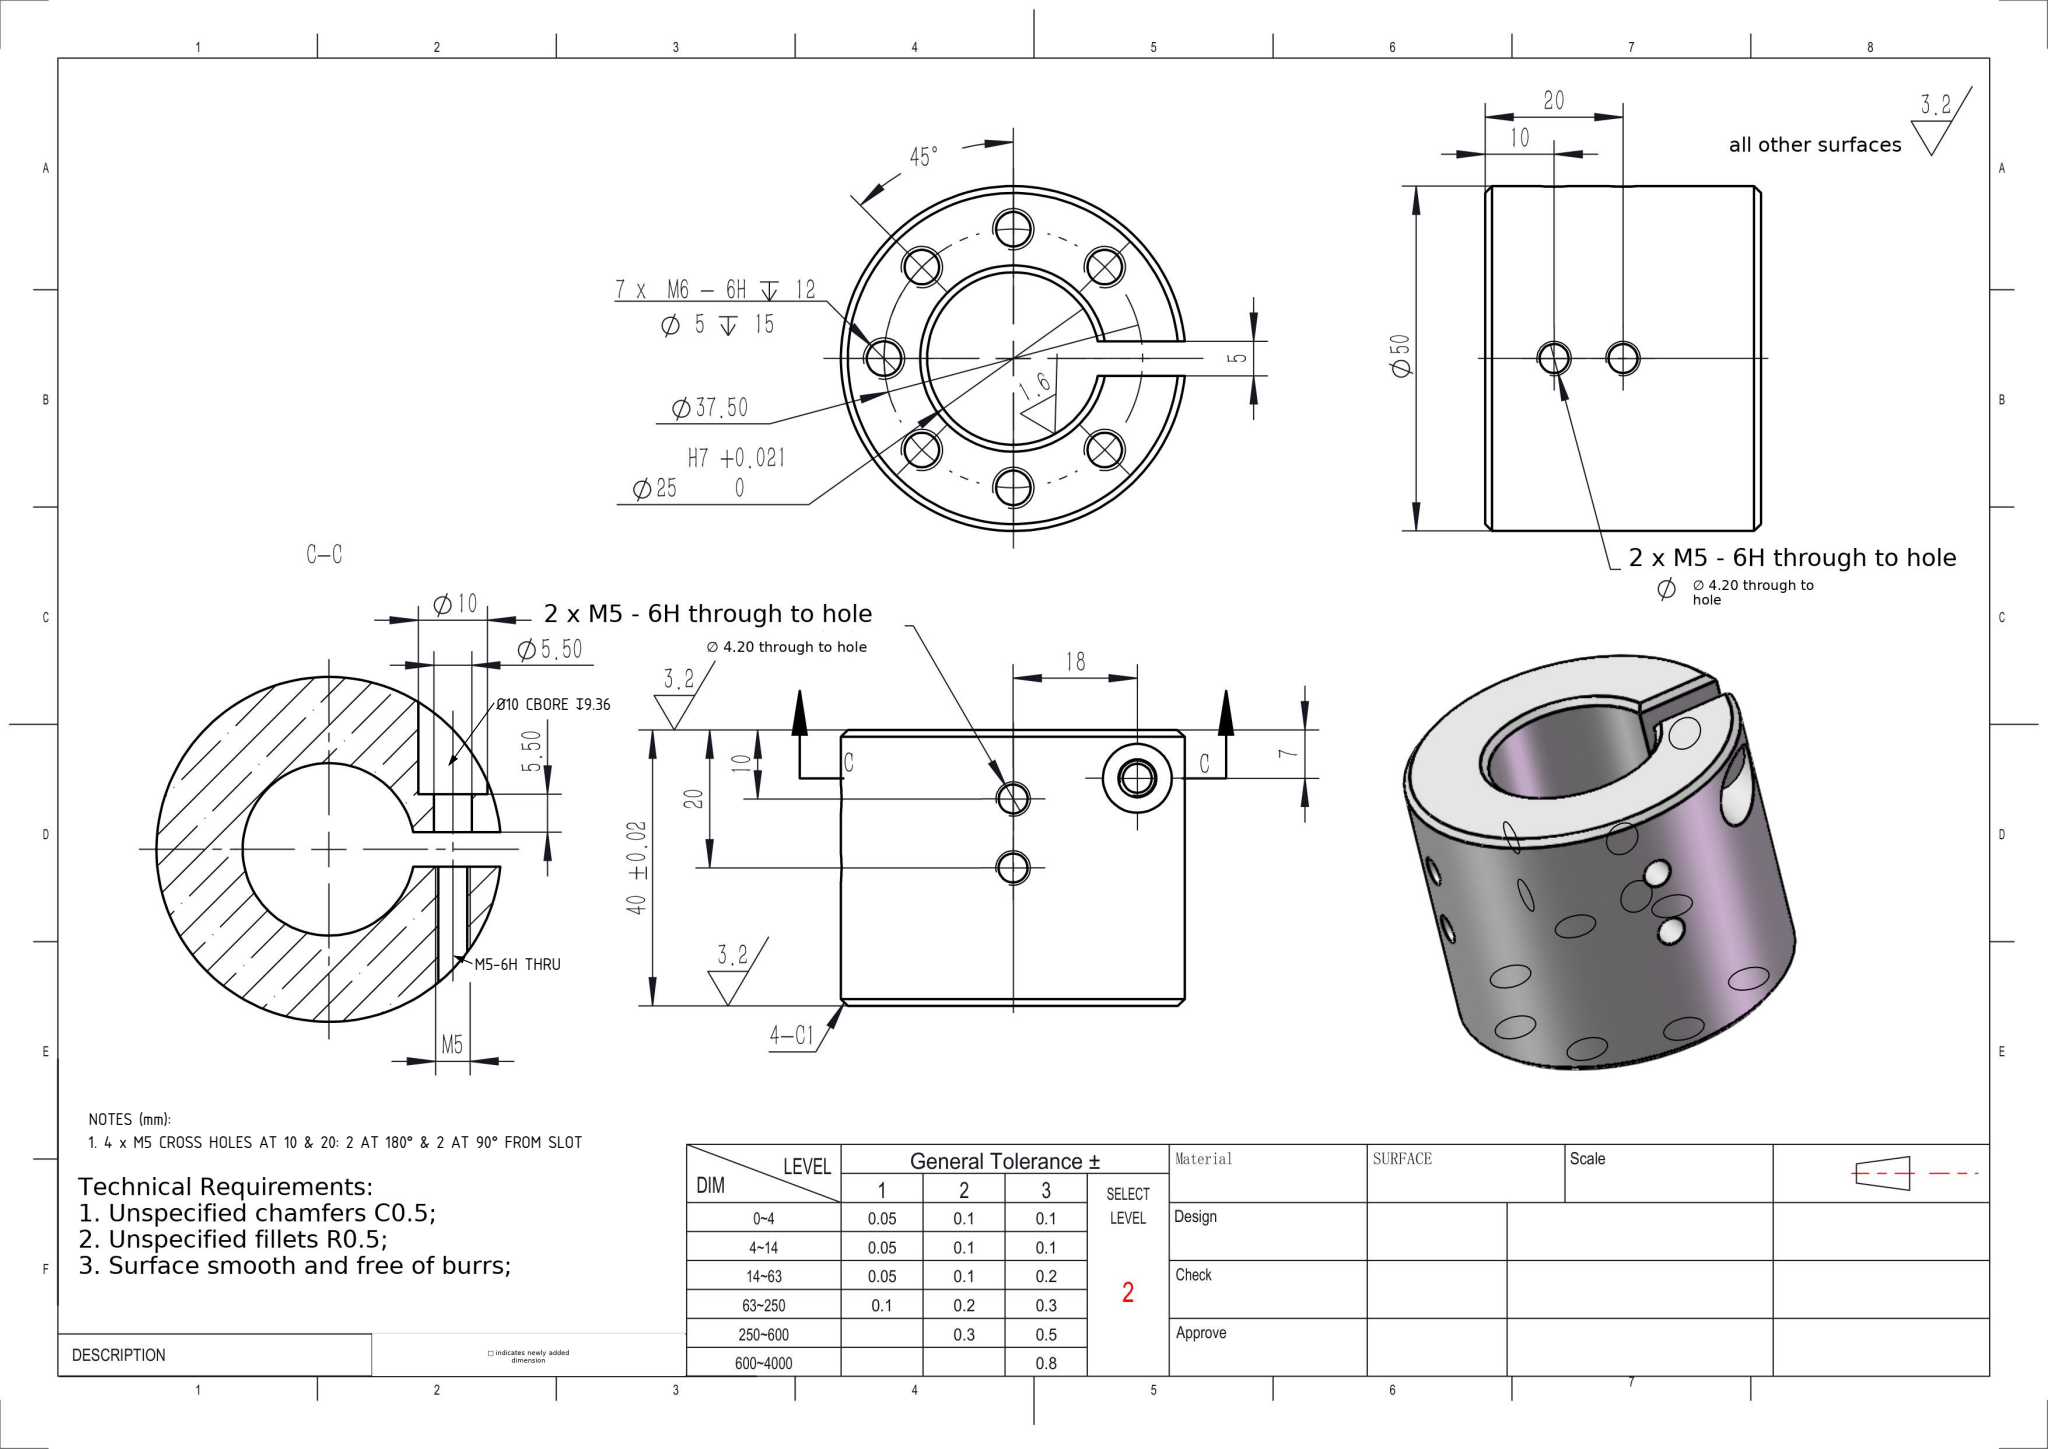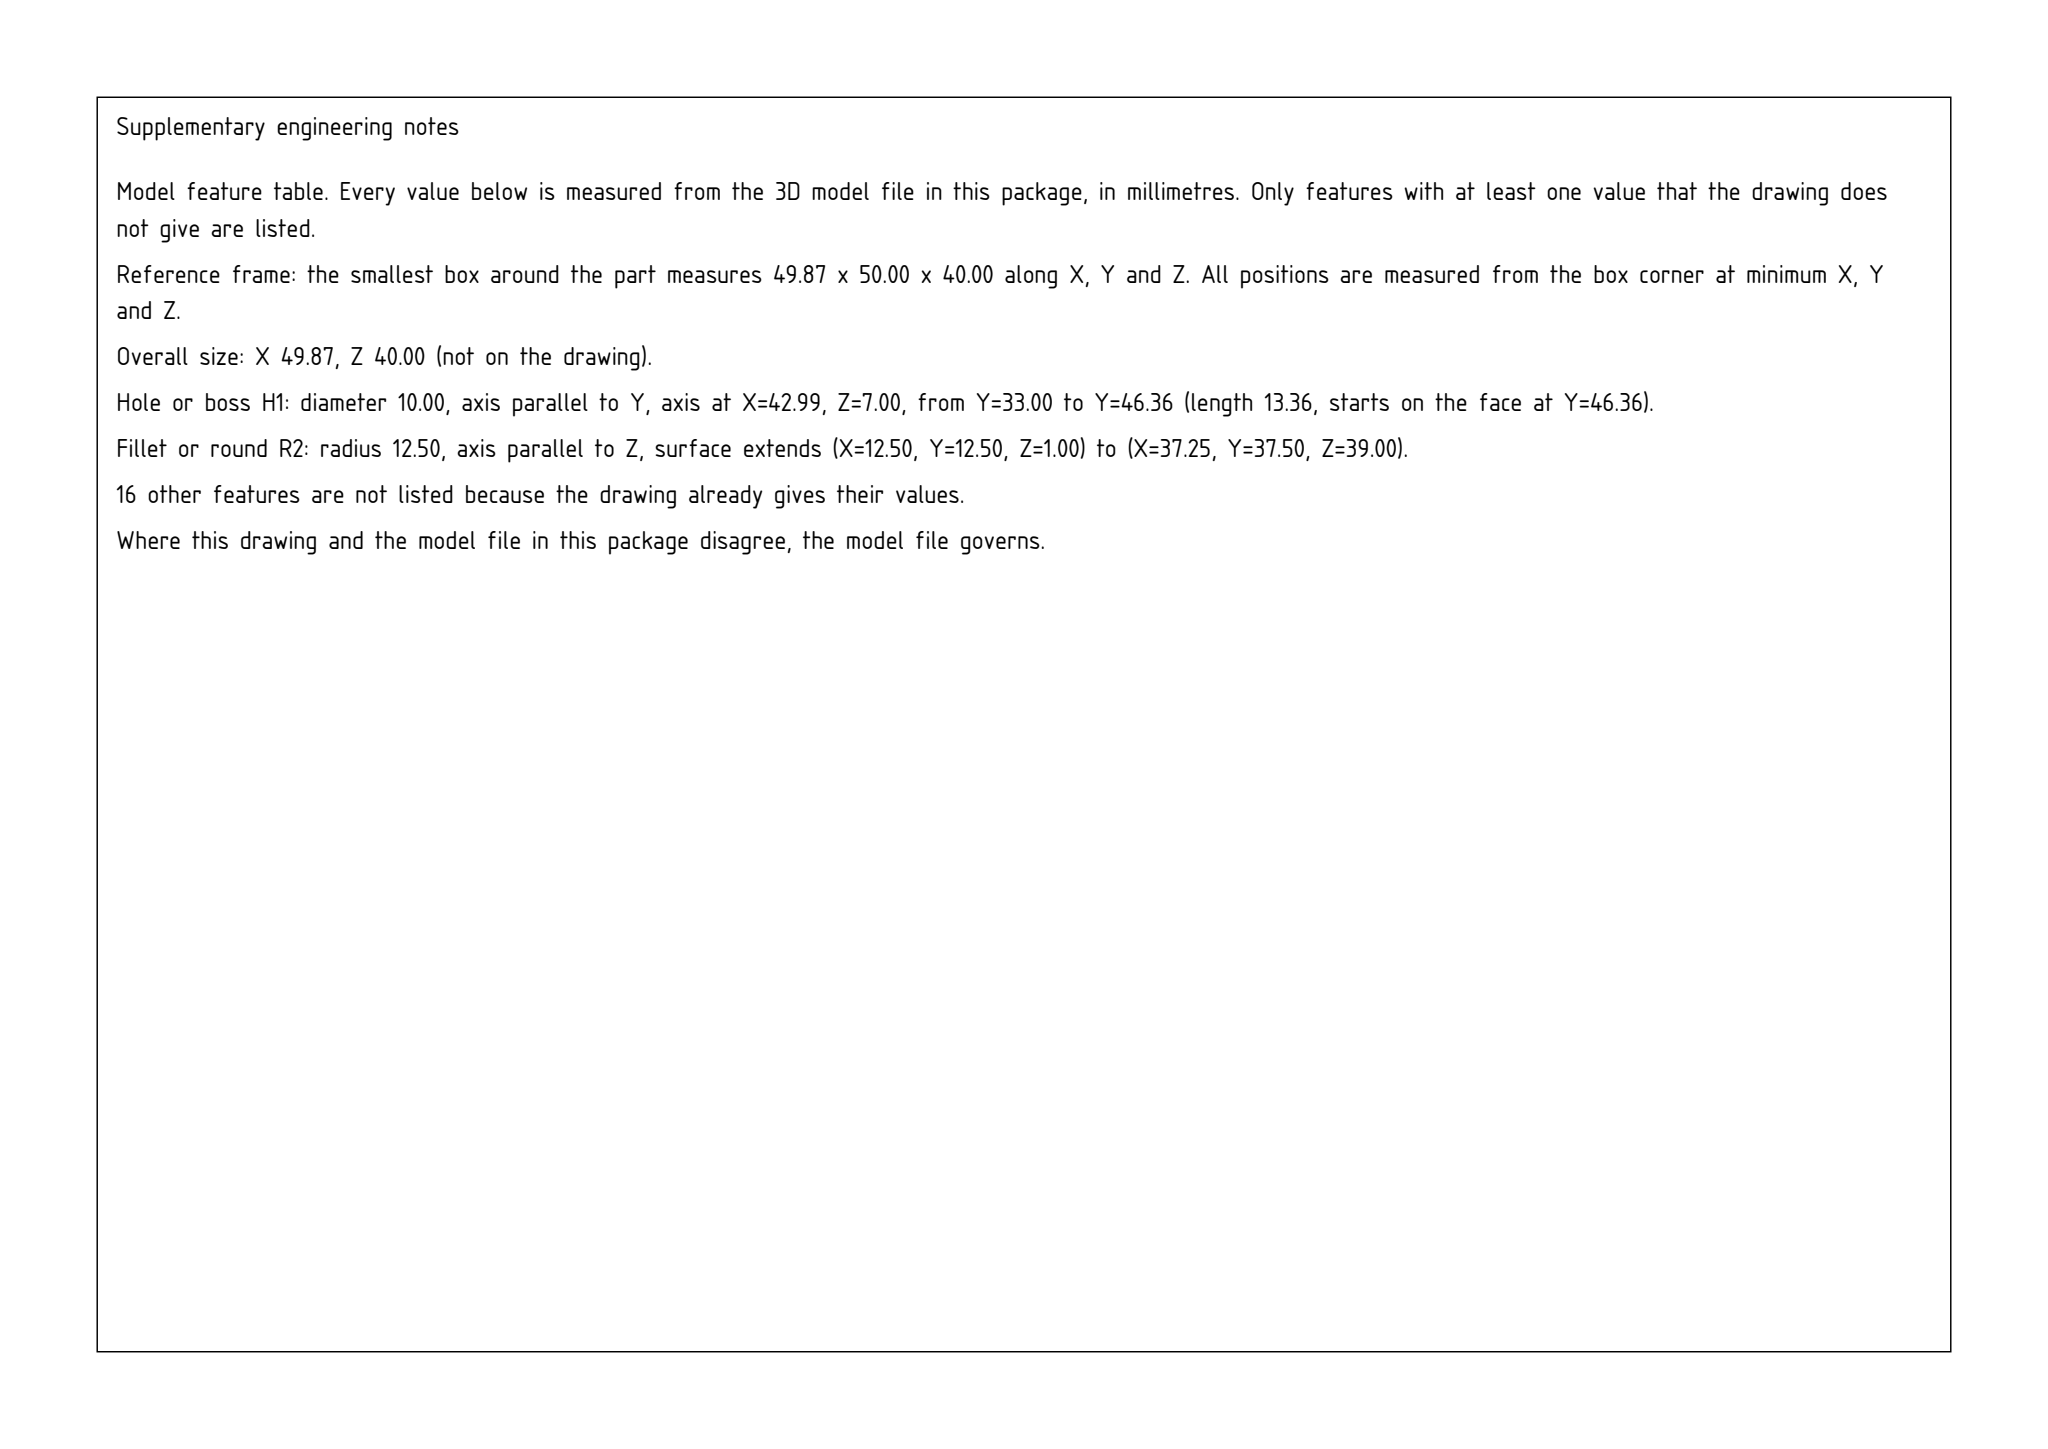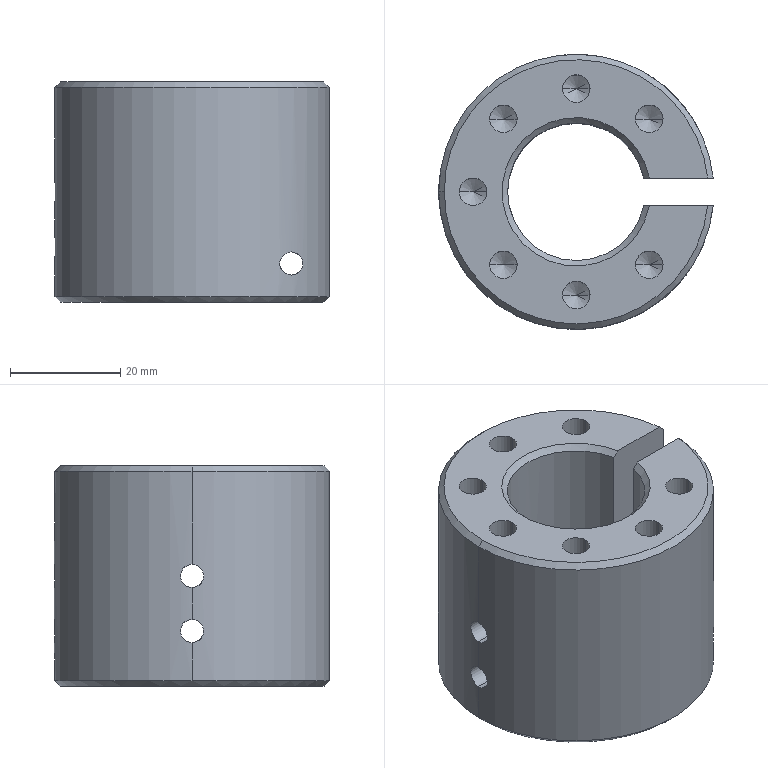Part | SolidWorks | mm | 1 solid | 59 faces | box 49.87 x 50 x 40 mm | volume 52296 mm3 | cylinder 32 | cone 20 | plane 7 | commonest cylinder face diameters 5 x14 4.2 x10 5.5 x2 10 x2 25 x2 50 x2
Drawing notes:
4 x M5 CROSS HOLES AT 10 & 20: 2 AT 180° & 2 AT 90° FROM SLOT | from the solid: Ø4.2 holes: axis X at y=25 (slot CL plane, drilled opposite slot side) z=10 & z=20; axis Y at x=25 (90° to slot CL) z=10 & z=20; slot faces y=22.5/27.5 open toward +x
C-C: Ø10 C'BORE DP 9.36 FROM Ø50 OD AT SCREW CL | from the solid: Ø10 bore along Y at x=42.99, z=7; flat bottom plane y=33.0; OD Ø50 at x=42.99 gives y=42.36, so depth 42.36-33.0=9.36 (Ø5.50 then 5.50 to slot face y=27.5)
C-C: M5-6H THRU (14.86 THD AT CL) | from the solid: Ø4.2 tap drill along Y at x=42.99, z=7, length 14.86 at CL from slot face y=22.5 to OD y=7.64; no 118° drill point present for this hole = through
build123d program:
from build123d import *

# Parameters (mm, degrees)
SKETCH1_R                                         = 25
SKETCH1_R_2                                       = 12.5
BOSS_EXTRUDE1_DEPTH                               = 40
SKETCH2_W                                         = 25
SKETCH2_H                                         = 5
CUT_EXTRUDE1_DEPTH                                = 50
M6_TAPPED_HOLE1_D                                 = 5
M6_TAPPED_HOLE1_DEPTH                             = 15
M6_TAPPED_HOLE1_TIP                               = 1.502
HOLE_SIZE_ACCORDING_TO_HEX_SOCKET_HEA_D           = 5.5
HOLE_SIZE_ACCORDING_TO_HEX_SOCKET_HEA_DEPTH       = 22.5
HOLE_SIZE_ACCORDING_TO_HEX_SOCKET_HEA_CBORE_D     = 10
HOLE_SIZE_ACCORDING_TO_HEX_SOCKET_HEA_CBORE_DEPTH = 17
M5_TAPPED_HOLE1_D                                 = 4.2
SKETCH18_W                                        = 2.1
SKETCH18_H                                        = 25
M5_TAPPED_HOLE2_AT_2_COUNT                        = 2
M5_TAPPED_HOLE2_AT_2_PITCH                        = 10
M5_TAPPED_HOLE3_D                                 = 4.2
CHAMFER1_SIZE                                     = 1


with BuildPart() as part:
    # Sketch1 → Boss-Extrude1 (new body)
    with BuildSketch(Plane.XY):
        Circle(SKETCH1_R)
        Circle(SKETCH1_R_2, mode=Mode.SUBTRACT)
    extrude(amount=BOSS_EXTRUDE1_DEPTH)

    # Sketch2 → Cut-Extrude1 (cut)
    with BuildSketch(Plane.XY.offset(40)):
        with Locations((17.5, 0)):
            Rectangle(SKETCH2_W, SKETCH2_H)
    extrude(amount=-CUT_EXTRUDE1_DEPTH, mode=Mode.SUBTRACT)

    # M6 Tapped Hole1
    with Locations(Plane.XY.offset(40)):
        with Locations((0, 18.75), (13.258, 13.258), (13.258, -13.258), (0, -18.75), (-13.258, -13.258), (-18.75, 0), (-13.258, 13.258), (18.75, 0)):
            Hole(M6_TAPPED_HOLE1_D / 2, depth=M6_TAPPED_HOLE1_DEPTH)
            with Locations((0, 0, -(M6_TAPPED_HOLE1_DEPTH + M6_TAPPED_HOLE1_TIP / 2))):  # 118° drill point
                Cone(0, M6_TAPPED_HOLE1_D / 2, M6_TAPPED_HOLE1_TIP, mode=Mode.SUBTRACT)

    # Hole Size _ according to_ Hex Socket Hea
    with Locations(Plane(origin=(0, 25, 0), x_dir=(1, 0, 0), z_dir=(0, 1, 0))):
        with Locations((17.989, -7)):
            CounterBoreHole(HOLE_SIZE_ACCORDING_TO_HEX_SOCKET_HEA_D / 2, HOLE_SIZE_ACCORDING_TO_HEX_SOCKET_HEA_CBORE_D / 2, HOLE_SIZE_ACCORDING_TO_HEX_SOCKET_HEA_CBORE_DEPTH, depth=HOLE_SIZE_ACCORDING_TO_HEX_SOCKET_HEA_DEPTH)

    # M5 Tapped Hole1 (through all)
    with Locations(Plane(origin=(0, -2.5, 0), x_dir=(1, 0, 0), z_dir=(0, 1, 0))):
        with Locations((17.989, -7)):
            Hole(M5_TAPPED_HOLE1_D / 2)

    # Sketch18 → M5 Tapped Hole2 (revolve, cut)
    with BuildSketch(Plane(origin=(-0.01566, 0, 10), x_dir=(0, 0, -1), z_dir=(1, 0, 0))):
        with Locations((1.05, 12.5)):
            Rectangle(SKETCH18_W, SKETCH18_H)
    m5_tapped_hole2 = revolve(axis=Axis((-0.01566, -6.35, 10), (0, 1, 0)), mode=Mode.SUBTRACT)

    # M5 Tapped Hole2 at 2: M5 Tapped Hole2 ×2
    with Locations(*[Vector(-0.001566, 0, 1) * (i * M5_TAPPED_HOLE2_AT_2_PITCH) for i in range(1, M5_TAPPED_HOLE2_AT_2_COUNT)]):
        add(m5_tapped_hole2, mode=Mode.SUBTRACT)

    # M5 Tapped Hole3 (through all)
    with Locations(Plane(origin=(0, 0, 0), x_dir=(0, 0, -1), z_dir=(1, 0, 0))):
        with Locations((-20, 0), (-10, 0)):
            Hole(M5_TAPPED_HOLE3_D / 2)

    # Chamfer1
    chamfer1_edges = [part.edges().sort_by_distance(p)[0] for p in [
        (18.561, 2.5, 0),
        (18.561, -2.5, 0),
        (-25, 0, 0),
        (-25, 0, 40),
        (-12.5, 0, 0),
        (-12.5, 0, 40),
    ]]
    chamfer(chamfer1_edges, length=CHAMFER1_SIZE)


solid = part.part